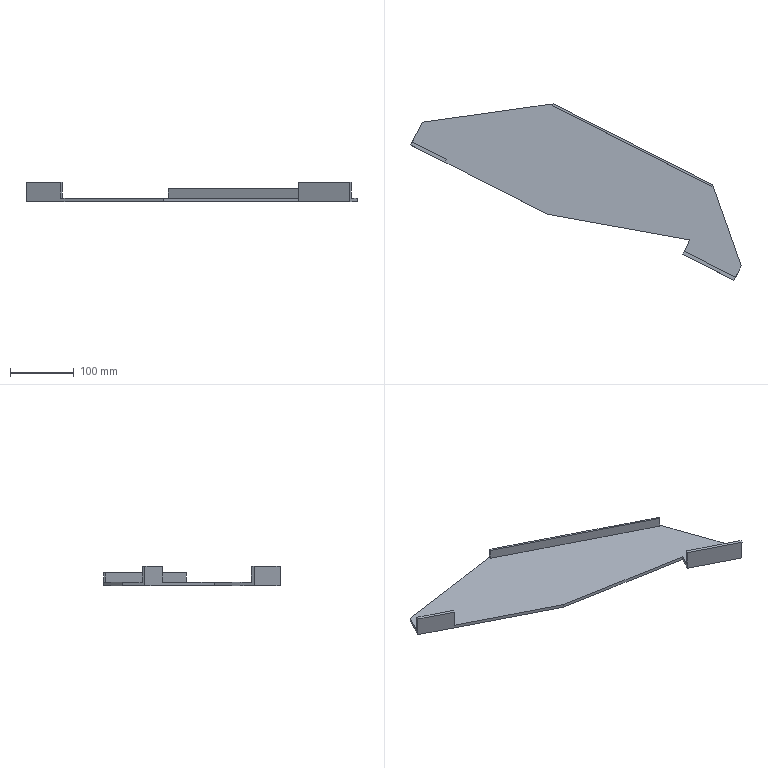Component | SolidWorks | Part18-1 | 2 solids | 22 faces | box 517.58 x 276.19 x 30 mm | volume 338137 mm3 | plane 22
build123d program:
from build123d import *

# Parameters (mm, degrees)
BOSS_EXTRUDE1_DEPTH = 5
SKETCH2_W           = 90
SKETCH2_H           = 30
BOSS_EXTRUDE2_DEPTH = 5
SKETCH3_W           = 280
SKETCH3_H           = 15
BOSS_EXTRUDE3_DEPTH = 3
SKETCH4_W           = 60
SKETCH4_H           = 25
BOSS_EXTRUDE4_DEPTH = 5


with BuildPart() as part:
    # Sketch1 → Boss-Extrude1 (new body)
    with BuildSketch(Plane.XY):
        Polygon((-37.937, 0), (-37.937, 20), (59.702, 113.229), (339.702, 113.229), (509.386, -5), (509.386, -45), (269.386, -45), (52.063, 20), (52.063, 0), align=None)
    extrude(amount=BOSS_EXTRUDE1_DEPTH)

    # Sketch2 → Boss-Extrude2 (add)
    with BuildSketch(Plane(origin=(0, 0, 0), x_dir=(-1, 0, 0), z_dir=(0, -1, 0))):
        with Locations((-7.063, 10)):
            Rectangle(SKETCH2_W, SKETCH2_H)
    extrude(amount=BOSS_EXTRUDE2_DEPTH)

    # Sketch4 → Boss-Extrude4 (add)
    with BuildSketch(Plane(origin=(0, -45, 0), x_dir=(-1, 0, 0), z_dir=(0, -1, 0))):
        with Locations((-479.386, 12.5)):
            Rectangle(SKETCH4_W, SKETCH4_H)
    extrude(amount=-BOSS_EXTRUDE4_DEPTH)


with BuildPart() as body_2:
    # Sketch3 → Boss-Extrude3 (new body)
    with BuildSketch(Plane(origin=(0, 113.229, 0), x_dir=(1, 0, 0), z_dir=(0, 1, 0))):
        with Locations((199.702, 7.5)):
            Rectangle(SKETCH3_W, SKETCH3_H)
    extrude(amount=-BOSS_EXTRUDE3_DEPTH)


solid = Compound([part.part, body_2.part])

# Placed as in the assembly
solid = solid.moved(Location((298.812, -1061.476, 1167.971), (-180, 0, -153.121)))
STEP:
#1=CARTESIAN_POINT('',(11.683,-36.751,45.983));
#2=VERTEX_POINT('',#1);
#3=CARTESIAN_POINT('',(1.85,-31.768,45.983));
#4=VERTEX_POINT('',#3);
#5=CARTESIAN_POINT('',(1.85,-31.768,45.983));
#6=DIRECTION('',(-0.892,0.4521,0.));
#7=VECTOR('',#6,39.37);
#8=LINE('',#5,#7);
#9=EDGE_CURVE('',#2,#4,#8,.T.);
#10=ORIENTED_EDGE('',*,*,#9,.F.);
#11=CARTESIAN_POINT('',(11.63,-36.857,45.983));
#12=VERTEX_POINT('',#11);
#13=CARTESIAN_POINT('',(11.63,-36.857,45.983));
#14=DIRECTION('',(0.4521,0.892,0.));
#15=VECTOR('',#14,39.37);
#16=LINE('',#13,#15);
#17=EDGE_CURVE('',#12,#2,#16,.T.);
#18=ORIENTED_EDGE('',*,*,#17,.F.);
#19=CARTESIAN_POINT('',(1.797,-31.873,45.983));
#20=VERTEX_POINT('',#19);
#21=CARTESIAN_POINT('',(1.797,-31.873,45.983));
#22=DIRECTION('',(-0.892,0.4521,0.));
#23=VECTOR('',#22,39.37);
#24=LINE('',#21,#23);
#25=EDGE_CURVE('',#12,#20,#24,.T.);
#26=ORIENTED_EDGE('',*,*,#25,.T.);
#27=CARTESIAN_POINT('',(1.797,-31.873,45.983));
#28=DIRECTION('',(0.4521,0.892,0.));
#29=VECTOR('',#28,39.37);
#30=LINE('',#27,#29);
#31=EDGE_CURVE('',#20,#4,#30,.T.);
#32=ORIENTED_EDGE('',*,*,#31,.T.);
#33=EDGE_LOOP('',(#10,#18,#26,#32));
#34=FACE_OUTER_BOUND('',#33,.T.);
#35=CARTESIAN_POINT('',(1.797,-31.873,45.983));
#36=DIRECTION('',(0.,0.,-1.));
#37=DIRECTION('',(-0.892,0.4521,0.));
#38=AXIS2_PLACEMENT_3D('',#35,#36,#37);
#39=PLANE('',#38);
#40=ADVANCED_FACE('',(#34),#39,.T.);
#41=CARTESIAN_POINT('',(11.683,-36.751,46.574));
#42=VERTEX_POINT('',#41);
#43=CARTESIAN_POINT('',(11.683,-36.751,45.983));
#44=DIRECTION('',(0.,0.,-1.));
#45=VECTOR('',#44,39.37);
#46=LINE('',#43,#45);
#47=EDGE_CURVE('',#42,#2,#46,.T.);
#48=ORIENTED_EDGE('',*,*,#47,.F.);
#49=CARTESIAN_POINT('',(11.63,-36.857,46.574));
#50=VERTEX_POINT('',#49);
#51=CARTESIAN_POINT('',(11.63,-36.857,46.574));
#52=DIRECTION('',(0.4521,0.892,0.));
#53=VECTOR('',#52,39.37);
#54=LINE('',#51,#53);
#55=EDGE_CURVE('',#50,#42,#54,.T.);
#56=ORIENTED_EDGE('',*,*,#55,.F.);
#57=CARTESIAN_POINT('',(11.63,-36.857,45.983));
#58=DIRECTION('',(0.,0.,-1.));
#59=VECTOR('',#58,39.37);
#60=LINE('',#57,#59);
#61=EDGE_CURVE('',#50,#12,#60,.T.);
#62=ORIENTED_EDGE('',*,*,#61,.T.);
#63=ORIENTED_EDGE('',*,*,#17,.T.);
#64=EDGE_LOOP('',(#48,#56,#62,#63));
#65=FACE_OUTER_BOUND('',#64,.T.);
#66=CARTESIAN_POINT('',(11.63,-36.857,45.983));
#67=DIRECTION('',(0.892,-0.4521,-0.));
#68=DIRECTION('',(0.,0.,-1.));
#69=AXIS2_PLACEMENT_3D('',#66,#67,#68);
#70=PLANE('',#69);
#71=ADVANCED_FACE('',(#65),#70,.T.);
#72=CARTESIAN_POINT('',(1.85,-31.768,46.574));
#73=VERTEX_POINT('',#72);
#74=CARTESIAN_POINT('',(11.683,-36.751,46.574));
#75=DIRECTION('',(0.892,-0.4521,-0.));
#76=VECTOR('',#75,39.37);
#77=LINE('',#74,#76);
#78=EDGE_CURVE('',#73,#42,#77,.T.);
#79=ORIENTED_EDGE('',*,*,#78,.F.);
#80=CARTESIAN_POINT('',(1.797,-31.873,46.574));
#81=VERTEX_POINT('',#80);
#82=CARTESIAN_POINT('',(1.797,-31.873,46.574));
#83=DIRECTION('',(0.4521,0.892,0.));
#84=VECTOR('',#83,39.37);
#85=LINE('',#82,#84);
#86=EDGE_CURVE('',#81,#73,#85,.T.);
#87=ORIENTED_EDGE('',*,*,#86,.F.);
#88=CARTESIAN_POINT('',(11.63,-36.857,46.574));
#89=DIRECTION('',(0.892,-0.4521,-0.));
#90=VECTOR('',#89,39.37);
#91=LINE('',#88,#90);
#92=EDGE_CURVE('',#81,#50,#91,.T.);
#93=ORIENTED_EDGE('',*,*,#92,.T.);
#94=ORIENTED_EDGE('',*,*,#55,.T.);
#95=EDGE_LOOP('',(#79,#87,#93,#94));
#96=FACE_OUTER_BOUND('',#95,.T.);
#97=CARTESIAN_POINT('',(11.63,-36.857,46.574));
#98=DIRECTION('',(-0.,-0.,1.));
#99=DIRECTION('',(0.892,-0.4521,-0.));
#100=AXIS2_PLACEMENT_3D('',#97,#98,#99);
#101=PLANE('',#100);
#102=ADVANCED_FACE('',(#96),#101,.T.);
#103=CARTESIAN_POINT('',(1.85,-31.768,46.574));
#104=DIRECTION('',(-0.,-0.,1.));
#105=VECTOR('',#104,39.37);
#106=LINE('',#103,#105);
#107=EDGE_CURVE('',#4,#73,#106,.T.);
#108=ORIENTED_EDGE('',*,*,#107,.F.);
#109=ORIENTED_EDGE('',*,*,#31,.F.);
#110=CARTESIAN_POINT('',(1.797,-31.873,46.574));
#111=DIRECTION('',(-0.,-0.,1.));
#112=VECTOR('',#111,39.37);
#113=LINE('',#110,#112);
#114=EDGE_CURVE('',#20,#81,#113,.T.);
#115=ORIENTED_EDGE('',*,*,#114,.T.);
#116=ORIENTED_EDGE('',*,*,#86,.T.);
#117=EDGE_LOOP('',(#108,#109,#115,#116));
#118=FACE_OUTER_BOUND('',#117,.T.);
#119=CARTESIAN_POINT('',(1.797,-31.873,46.574));
#120=DIRECTION('',(-0.892,0.4521,0.));
#121=DIRECTION('',(-0.,-0.,1.));
#122=AXIS2_PLACEMENT_3D('',#119,#120,#121);
#123=PLANE('',#122);
#124=ADVANCED_FACE('',(#118),#123,.T.);
#125=ORIENTED_EDGE('',*,*,#25,.F.);
#126=ORIENTED_EDGE('',*,*,#61,.F.);
#127=ORIENTED_EDGE('',*,*,#92,.F.);
#128=ORIENTED_EDGE('',*,*,#114,.F.);
#129=EDGE_LOOP('',(#125,#126,#127,#128));
#130=FACE_OUTER_BOUND('',#129,.T.);
#131=CARTESIAN_POINT('',(13.726,-37.919,45.983));
#132=DIRECTION('',(-0.4521,-0.892,-0.));
#133=DIRECTION('',(-0.,-0.,1.));
#134=AXIS2_PLACEMENT_3D('',#131,#132,#133);
#135=PLANE('',#134);
#136=ADVANCED_FACE('',(#130),#135,.T.);
#137=ORIENTED_EDGE('',*,*,#9,.T.);
#138=ORIENTED_EDGE('',*,*,#107,.T.);
#139=ORIENTED_EDGE('',*,*,#78,.T.);
#140=ORIENTED_EDGE('',*,*,#47,.T.);
#141=EDGE_LOOP('',(#137,#138,#139,#140));
#142=FACE_OUTER_BOUND('',#141,.T.);
#143=CARTESIAN_POINT('',(13.78,-37.814,45.983));
#144=DIRECTION('',(-0.4521,-0.892,-0.));
#145=DIRECTION('',(-0.,-0.,1.));
#146=AXIS2_PLACEMENT_3D('',#143,#144,#145);
#147=PLANE('',#146);
#148=ADVANCED_FACE('',(#142),#147,.F.);
#149=CLOSED_SHELL('',(#40,#71,#102,#124,#136,#148));
#150=MANIFOLD_SOLID_BREP('',#149);
#151=CARTESIAN_POINT('',(9.936,-40.864,45.983));
#152=VERTEX_POINT('',#151);
#153=CARTESIAN_POINT('',(10.292,-40.161,45.983));
#154=VERTEX_POINT('',#153);
#155=CARTESIAN_POINT('',(9.936,-40.864,45.983));
#156=DIRECTION('',(0.4521,0.892,0.));
#157=VECTOR('',#156,39.37);
#158=LINE('',#155,#157);
#159=EDGE_CURVE('',#152,#154,#158,.T.);
#160=ORIENTED_EDGE('',*,*,#159,.T.);
#161=CARTESIAN_POINT('',(10.292,-40.161,45.786));
#162=VERTEX_POINT('',#161);
#163=CARTESIAN_POINT('',(10.292,-40.161,45.786));
#164=DIRECTION('',(-0.,-0.,1.));
#165=VECTOR('',#164,39.37);
#166=LINE('',#163,#165);
#167=EDGE_CURVE('',#162,#154,#166,.T.);
#168=ORIENTED_EDGE('',*,*,#167,.F.);
#169=CARTESIAN_POINT('',(9.847,-41.039,45.786));
#170=VERTEX_POINT('',#169);
#171=CARTESIAN_POINT('',(9.936,-40.864,45.786));
#172=DIRECTION('',(0.4521,0.892,0.));
#173=VECTOR('',#172,39.37);
#174=LINE('',#171,#173);
#175=EDGE_CURVE('',#170,#162,#174,.T.);
#176=ORIENTED_EDGE('',*,*,#175,.F.);
#177=CARTESIAN_POINT('',(9.847,-41.039,46.967));
#178=VERTEX_POINT('',#177);
#179=CARTESIAN_POINT('',(9.847,-41.039,45.786));
#180=DIRECTION('',(0.,0.,-1.));
#181=VECTOR('',#180,39.37);
#182=LINE('',#179,#181);
#183=EDGE_CURVE('',#178,#170,#182,.T.);
#184=ORIENTED_EDGE('',*,*,#183,.F.);
#185=CARTESIAN_POINT('',(9.936,-40.864,46.967));
#186=VERTEX_POINT('',#185);
#187=CARTESIAN_POINT('',(9.847,-41.039,46.967));
#188=DIRECTION('',(0.4521,0.892,0.));
#189=VECTOR('',#188,39.37);
#190=LINE('',#187,#189);
#191=EDGE_CURVE('',#178,#186,#190,.T.);
#192=ORIENTED_EDGE('',*,*,#191,.T.);
#193=CARTESIAN_POINT('',(9.936,-40.864,45.786));
#194=DIRECTION('',(0.,0.,-1.));
#195=VECTOR('',#194,39.37);
#196=LINE('',#193,#195);
#197=EDGE_CURVE('',#186,#152,#196,.T.);
#198=ORIENTED_EDGE('',*,*,#197,.T.);
#199=EDGE_LOOP('',(#160,#168,#176,#184,#192,#198));
#200=FACE_OUTER_BOUND('',#199,.T.);
#201=CARTESIAN_POINT('',(9.936,-40.864,45.786));
#202=DIRECTION('',(0.892,-0.4521,-0.));
#203=DIRECTION('',(0.,0.,-1.));
#204=AXIS2_PLACEMENT_3D('',#201,#202,#203);
#205=PLANE('',#204);
#206=ADVANCED_FACE('',(#200),#205,.F.);
#207=CARTESIAN_POINT('',(1.503,-38.576,45.983));
#208=VERTEX_POINT('',#207);
#209=CARTESIAN_POINT('',(10.292,-40.161,45.983));
#210=DIRECTION('',(-0.9841,0.1775,0.));
#211=VECTOR('',#210,39.37);
#212=LINE('',#209,#211);
#213=EDGE_CURVE('',#154,#208,#212,.T.);
#214=ORIENTED_EDGE('',*,*,#213,.T.);
#215=CARTESIAN_POINT('',(1.503,-38.576,45.786));
#216=VERTEX_POINT('',#215);
#217=CARTESIAN_POINT('',(1.503,-38.576,45.786));
#218=DIRECTION('',(-0.,-0.,1.));
#219=VECTOR('',#218,39.37);
#220=LINE('',#217,#219);
#221=EDGE_CURVE('',#216,#208,#220,.T.);
#222=ORIENTED_EDGE('',*,*,#221,.F.);
#223=CARTESIAN_POINT('',(10.292,-40.161,45.786));
#224=DIRECTION('',(-0.9841,0.1775,0.));
#225=VECTOR('',#224,39.37);
#226=LINE('',#223,#225);
#227=EDGE_CURVE('',#162,#216,#226,.T.);
#228=ORIENTED_EDGE('',*,*,#227,.F.);
#229=ORIENTED_EDGE('',*,*,#167,.T.);
#230=EDGE_LOOP('',(#214,#222,#228,#229));
#231=FACE_OUTER_BOUND('',#230,.T.);
#232=CARTESIAN_POINT('',(10.292,-40.161,45.786));
#233=DIRECTION('',(0.1775,0.9841,0.));
#234=DIRECTION('',(0.9841,-0.1775,-0.));
#235=AXIS2_PLACEMENT_3D('',#232,#233,#234);
#236=PLANE('',#235);
#237=ADVANCED_FACE('',(#231),#236,.F.);
#238=CARTESIAN_POINT('',(-4.818,-35.372,45.983));
#239=VERTEX_POINT('',#238);
#240=CARTESIAN_POINT('',(1.503,-38.576,45.983));
#241=DIRECTION('',(-0.892,0.4521,0.));
#242=VECTOR('',#241,39.37);
#243=LINE('',#240,#242);
#244=EDGE_CURVE('',#208,#239,#243,.T.);
#245=ORIENTED_EDGE('',*,*,#244,.T.);
#246=CARTESIAN_POINT('',(-4.818,-35.372,46.967));
#247=VERTEX_POINT('',#246);
#248=CARTESIAN_POINT('',(-4.818,-35.372,46.967));
#249=DIRECTION('',(-0.,-0.,1.));
#250=VECTOR('',#249,39.37);
#251=LINE('',#248,#250);
#252=EDGE_CURVE('',#239,#247,#251,.T.);
#253=ORIENTED_EDGE('',*,*,#252,.T.);
#254=CARTESIAN_POINT('',(-6.925,-34.304,46.967));
#255=VERTEX_POINT('',#254);
#256=CARTESIAN_POINT('',(-6.925,-34.304,46.967));
#257=DIRECTION('',(-0.892,0.4521,0.));
#258=VECTOR('',#257,39.37);
#259=LINE('',#256,#258);
#260=EDGE_CURVE('',#247,#255,#259,.T.);
#261=ORIENTED_EDGE('',*,*,#260,.T.);
#262=CARTESIAN_POINT('',(-6.925,-34.304,45.786));
#263=VERTEX_POINT('',#262);
#264=CARTESIAN_POINT('',(-6.925,-34.304,45.786));
#265=DIRECTION('',(-0.,-0.,1.));
#266=VECTOR('',#265,39.37);
#267=LINE('',#264,#266);
#268=EDGE_CURVE('',#263,#255,#267,.T.);
#269=ORIENTED_EDGE('',*,*,#268,.F.);
#270=CARTESIAN_POINT('',(1.503,-38.576,45.786));
#271=DIRECTION('',(-0.892,0.4521,0.));
#272=VECTOR('',#271,39.37);
#273=LINE('',#270,#272);
#274=EDGE_CURVE('',#216,#263,#273,.T.);
#275=ORIENTED_EDGE('',*,*,#274,.F.);
#276=ORIENTED_EDGE('',*,*,#221,.T.);
#277=EDGE_LOOP('',(#245,#253,#261,#269,#275,#276));
#278=FACE_OUTER_BOUND('',#277,.T.);
#279=CARTESIAN_POINT('',(1.503,-38.576,45.786));
#280=DIRECTION('',(0.4521,0.892,0.));
#281=DIRECTION('',(0.,0.,-1.));
#282=AXIS2_PLACEMENT_3D('',#279,#280,#281);
#283=PLANE('',#282);
#284=ADVANCED_FACE('',(#278),#283,.F.);
#285=ORIENTED_EDGE('',*,*,#268,.T.);
#286=CARTESIAN_POINT('',(-6.836,-34.128,46.967));
#287=VERTEX_POINT('',#286);
#288=CARTESIAN_POINT('',(-6.836,-34.128,46.967));
#289=DIRECTION('',(-0.4521,-0.892,-0.));
#290=VECTOR('',#289,39.37);
#291=LINE('',#288,#290);
#292=EDGE_CURVE('',#287,#255,#291,.T.);
#293=ORIENTED_EDGE('',*,*,#292,.F.);
#294=CARTESIAN_POINT('',(-6.836,-34.128,45.983));
#295=VERTEX_POINT('',#294);
#296=CARTESIAN_POINT('',(-6.836,-34.128,45.983));
#297=DIRECTION('',(0.,0.,-1.));
#298=VECTOR('',#297,39.37);
#299=LINE('',#296,#298);
#300=EDGE_CURVE('',#287,#295,#299,.T.);
#301=ORIENTED_EDGE('',*,*,#300,.T.);
#302=CARTESIAN_POINT('',(-6.213,-32.899,45.983));
#303=VERTEX_POINT('',#302);
#304=CARTESIAN_POINT('',(-6.925,-34.304,45.983));
#305=DIRECTION('',(0.4521,0.892,0.));
#306=VECTOR('',#305,39.37);
#307=LINE('',#304,#306);
#308=EDGE_CURVE('',#295,#303,#307,.T.);
#309=ORIENTED_EDGE('',*,*,#308,.T.);
#310=CARTESIAN_POINT('',(-6.213,-32.899,45.786));
#311=VERTEX_POINT('',#310);
#312=CARTESIAN_POINT('',(-6.213,-32.899,45.786));
#313=DIRECTION('',(-0.,-0.,1.));
#314=VECTOR('',#313,39.37);
#315=LINE('',#312,#314);
#316=EDGE_CURVE('',#311,#303,#315,.T.);
#317=ORIENTED_EDGE('',*,*,#316,.F.);
#318=CARTESIAN_POINT('',(-6.925,-34.304,45.786));
#319=DIRECTION('',(0.4521,0.892,0.));
#320=VECTOR('',#319,39.37);
#321=LINE('',#318,#320);
#322=EDGE_CURVE('',#263,#311,#321,.T.);
#323=ORIENTED_EDGE('',*,*,#322,.F.);
#324=EDGE_LOOP('',(#285,#293,#301,#309,#317,#323));
#325=FACE_OUTER_BOUND('',#324,.T.);
#326=CARTESIAN_POINT('',(-6.925,-34.304,45.786));
#327=DIRECTION('',(0.892,-0.4521,-0.));
#328=DIRECTION('',(0.,0.,-1.));
#329=AXIS2_PLACEMENT_3D('',#326,#327,#328);
#330=PLANE('',#329);
#331=ADVANCED_FACE('',(#325),#330,.F.);
#332=CARTESIAN_POINT('',(1.85,-31.768,45.983));
#333=VERTEX_POINT('',#332);
#334=CARTESIAN_POINT('',(-6.213,-32.899,45.983));
#335=DIRECTION('',(0.9903,0.139,0.));
#336=VECTOR('',#335,39.37);
#337=LINE('',#334,#336);
#338=EDGE_CURVE('',#303,#333,#337,.T.);
#339=ORIENTED_EDGE('',*,*,#338,.T.);
#340=CARTESIAN_POINT('',(1.85,-31.768,45.786));
#341=VERTEX_POINT('',#340);
#342=CARTESIAN_POINT('',(1.85,-31.768,45.786));
#343=DIRECTION('',(-0.,-0.,1.));
#344=VECTOR('',#343,39.37);
#345=LINE('',#342,#344);
#346=EDGE_CURVE('',#341,#333,#345,.T.);
#347=ORIENTED_EDGE('',*,*,#346,.F.);
#348=CARTESIAN_POINT('',(-6.213,-32.899,45.786));
#349=DIRECTION('',(0.9903,0.139,0.));
#350=VECTOR('',#349,39.37);
#351=LINE('',#348,#350);
#352=EDGE_CURVE('',#311,#341,#351,.T.);
#353=ORIENTED_EDGE('',*,*,#352,.F.);
#354=ORIENTED_EDGE('',*,*,#316,.T.);
#355=EDGE_LOOP('',(#339,#347,#353,#354));
#356=FACE_OUTER_BOUND('',#355,.T.);
#357=CARTESIAN_POINT('',(-6.213,-32.899,45.786));
#358=DIRECTION('',(0.139,-0.9903,-0.));
#359=DIRECTION('',(-0.9903,-0.139,-0.));
#360=AXIS2_PLACEMENT_3D('',#357,#358,#359);
#361=PLANE('',#360);
#362=ADVANCED_FACE('',(#356),#361,.F.);
#363=CARTESIAN_POINT('',(11.683,-36.751,45.983));
#364=VERTEX_POINT('',#363);
#365=CARTESIAN_POINT('',(11.683,-36.751,45.983));
#366=DIRECTION('',(0.892,-0.4521,-0.));
#367=VECTOR('',#366,39.37);
#368=LINE('',#365,#367);
#369=EDGE_CURVE('',#333,#364,#368,.T.);
#370=ORIENTED_EDGE('',*,*,#369,.T.);
#371=CARTESIAN_POINT('',(11.683,-36.751,45.786));
#372=VERTEX_POINT('',#371);
#373=CARTESIAN_POINT('',(11.683,-36.751,45.786));
#374=DIRECTION('',(-0.,-0.,1.));
#375=VECTOR('',#374,39.37);
#376=LINE('',#373,#375);
#377=EDGE_CURVE('',#372,#364,#376,.T.);
#378=ORIENTED_EDGE('',*,*,#377,.F.);
#379=CARTESIAN_POINT('',(11.683,-36.751,45.786));
#380=DIRECTION('',(0.892,-0.4521,-0.));
#381=VECTOR('',#380,39.37);
#382=LINE('',#379,#381);
#383=EDGE_CURVE('',#341,#372,#382,.T.);
#384=ORIENTED_EDGE('',*,*,#383,.F.);
#385=ORIENTED_EDGE('',*,*,#346,.T.);
#386=EDGE_LOOP('',(#370,#378,#384,#385));
#387=FACE_OUTER_BOUND('',#386,.T.);
#388=CARTESIAN_POINT('',(11.683,-36.751,45.786));
#389=DIRECTION('',(-0.4521,-0.892,-0.));
#390=DIRECTION('',(-0.,-0.,1.));
#391=AXIS2_PLACEMENT_3D('',#388,#389,#390);
#392=PLANE('',#391);
#393=ADVANCED_FACE('',(#387),#392,.F.);
#394=CARTESIAN_POINT('',(13.452,-41.763,45.983));
#395=VERTEX_POINT('',#394);
#396=CARTESIAN_POINT('',(13.452,-41.763,45.983));
#397=DIRECTION('',(0.3329,-0.943,-0.));
#398=VECTOR('',#397,39.37);
#399=LINE('',#396,#398);
#400=EDGE_CURVE('',#364,#395,#399,.T.);
#401=ORIENTED_EDGE('',*,*,#400,.T.);
#402=CARTESIAN_POINT('',(13.452,-41.763,45.786));
#403=VERTEX_POINT('',#402);
#404=CARTESIAN_POINT('',(13.452,-41.763,45.786));
#405=DIRECTION('',(-0.,-0.,1.));
#406=VECTOR('',#405,39.37);
#407=LINE('',#404,#406);
#408=EDGE_CURVE('',#403,#395,#407,.T.);
#409=ORIENTED_EDGE('',*,*,#408,.F.);
#410=CARTESIAN_POINT('',(13.452,-41.763,45.786));
#411=DIRECTION('',(0.3329,-0.943,-0.));
#412=VECTOR('',#411,39.37);
#413=LINE('',#410,#412);
#414=EDGE_CURVE('',#372,#403,#413,.T.);
#415=ORIENTED_EDGE('',*,*,#414,.F.);
#416=ORIENTED_EDGE('',*,*,#377,.T.);
#417=EDGE_LOOP('',(#401,#409,#415,#416));
#418=FACE_OUTER_BOUND('',#417,.T.);
#419=CARTESIAN_POINT('',(13.452,-41.763,45.786));
#420=DIRECTION('',(-0.943,-0.3329,-0.));
#421=DIRECTION('',(-0.3329,0.943,0.));
#422=AXIS2_PLACEMENT_3D('',#419,#420,#421);
#423=PLANE('',#422);
#424=ADVANCED_FACE('',(#418),#423,.F.);
#425=CARTESIAN_POINT('',(13.096,-42.466,45.983));
#426=VERTEX_POINT('',#425);
#427=CARTESIAN_POINT('',(13.096,-42.466,45.983));
#428=DIRECTION('',(-0.4521,-0.892,-0.));
#429=VECTOR('',#428,39.37);
#430=LINE('',#427,#429);
#431=EDGE_CURVE('',#395,#426,#430,.T.);
#432=ORIENTED_EDGE('',*,*,#431,.T.);
#433=CARTESIAN_POINT('',(13.096,-42.466,46.967));
#434=VERTEX_POINT('',#433);
#435=CARTESIAN_POINT('',(13.096,-42.466,46.967));
#436=DIRECTION('',(-0.,-0.,1.));
#437=VECTOR('',#436,39.37);
#438=LINE('',#435,#437);
#439=EDGE_CURVE('',#426,#434,#438,.T.);
#440=ORIENTED_EDGE('',*,*,#439,.T.);
#441=CARTESIAN_POINT('',(13.007,-42.641,46.967));
#442=VERTEX_POINT('',#441);
#443=CARTESIAN_POINT('',(13.007,-42.641,46.967));
#444=DIRECTION('',(0.4521,0.892,0.));
#445=VECTOR('',#444,39.37);
#446=LINE('',#443,#445);
#447=EDGE_CURVE('',#442,#434,#446,.T.);
#448=ORIENTED_EDGE('',*,*,#447,.F.);
#449=CARTESIAN_POINT('',(13.007,-42.641,45.786));
#450=VERTEX_POINT('',#449);
#451=CARTESIAN_POINT('',(13.007,-42.641,46.967));
#452=DIRECTION('',(-0.,-0.,1.));
#453=VECTOR('',#452,39.37);
#454=LINE('',#451,#453);
#455=EDGE_CURVE('',#450,#442,#454,.T.);
#456=ORIENTED_EDGE('',*,*,#455,.F.);
#457=CARTESIAN_POINT('',(13.096,-42.466,45.786));
#458=DIRECTION('',(-0.4521,-0.892,-0.));
#459=VECTOR('',#458,39.37);
#460=LINE('',#457,#459);
#461=EDGE_CURVE('',#403,#450,#460,.T.);
#462=ORIENTED_EDGE('',*,*,#461,.F.);
#463=ORIENTED_EDGE('',*,*,#408,.T.);
#464=EDGE_LOOP('',(#432,#440,#448,#456,#462,#463));
#465=FACE_OUTER_BOUND('',#464,.T.);
#466=CARTESIAN_POINT('',(13.096,-42.466,45.786));
#467=DIRECTION('',(-0.892,0.4521,0.));
#468=DIRECTION('',(-0.,-0.,1.));
#469=AXIS2_PLACEMENT_3D('',#466,#467,#468);
#470=PLANE('',#469);
#471=ADVANCED_FACE('',(#465),#470,.F.);
#472=ORIENTED_EDGE('',*,*,#461,.T.);
#473=CARTESIAN_POINT('',(13.007,-42.641,45.786));
#474=DIRECTION('',(0.892,-0.4521,-0.));
#475=VECTOR('',#474,39.37);
#476=LINE('',#473,#475);
#477=EDGE_CURVE('',#170,#450,#476,.T.);
#478=ORIENTED_EDGE('',*,*,#477,.F.);
#479=ORIENTED_EDGE('',*,*,#175,.T.);
#480=ORIENTED_EDGE('',*,*,#227,.T.);
#481=ORIENTED_EDGE('',*,*,#274,.T.);
#482=ORIENTED_EDGE('',*,*,#322,.T.);
#483=ORIENTED_EDGE('',*,*,#352,.T.);
#484=ORIENTED_EDGE('',*,*,#383,.T.);
#485=ORIENTED_EDGE('',*,*,#414,.T.);
#486=EDGE_LOOP('',(#472,#478,#479,#480,#481,#482,#483,#484,#485));
#487=FACE_OUTER_BOUND('',#486,.T.);
#488=CARTESIAN_POINT('',(11.764,-41.79,45.786));
#489=DIRECTION('',(0.,0.,-1.));
#490=DIRECTION('',(-0.892,0.4521,0.));
#491=AXIS2_PLACEMENT_3D('',#488,#489,#490);
#492=PLANE('',#491);
#493=ADVANCED_FACE('',(#487),#492,.T.);
#494=CARTESIAN_POINT('',(-4.729,-35.196,45.983));
#495=VERTEX_POINT('',#494);
#496=CARTESIAN_POINT('',(-4.729,-35.196,45.983));
#497=DIRECTION('',(0.892,-0.4521,-0.));
#498=VECTOR('',#497,39.37);
#499=LINE('',#496,#498);
#500=EDGE_CURVE('',#295,#495,#499,.T.);
#501=ORIENTED_EDGE('',*,*,#500,.T.);
#502=CARTESIAN_POINT('',(-4.729,-35.196,45.983));
#503=DIRECTION('',(-0.4521,-0.892,-0.));
#504=VECTOR('',#503,39.37);
#505=LINE('',#502,#504);
#506=EDGE_CURVE('',#495,#239,#505,.T.);
#507=ORIENTED_EDGE('',*,*,#506,.T.);
#508=ORIENTED_EDGE('',*,*,#244,.F.);
#509=ORIENTED_EDGE('',*,*,#213,.F.);
#510=ORIENTED_EDGE('',*,*,#159,.F.);
#511=CARTESIAN_POINT('',(13.096,-42.466,45.983));
#512=DIRECTION('',(-0.892,0.4521,0.));
#513=VECTOR('',#512,39.37);
#514=LINE('',#511,#513);
#515=EDGE_CURVE('',#426,#152,#514,.T.);
#516=ORIENTED_EDGE('',*,*,#515,.F.);
#517=ORIENTED_EDGE('',*,*,#431,.F.);
#518=ORIENTED_EDGE('',*,*,#400,.F.);
#519=ORIENTED_EDGE('',*,*,#369,.F.);
#520=ORIENTED_EDGE('',*,*,#338,.F.);
#521=ORIENTED_EDGE('',*,*,#308,.F.);
#522=EDGE_LOOP('',(#501,#507,#508,#509,#510,#516,#517,#518,#519,#520,#521));
#523=FACE_OUTER_BOUND('',#522,.T.);
#524=CARTESIAN_POINT('',(11.764,-41.79,45.983));
#525=DIRECTION('',(0.,0.,-1.));
#526=DIRECTION('',(-0.892,0.4521,0.));
#527=AXIS2_PLACEMENT_3D('',#524,#525,#526);
#528=PLANE('',#527);
#529=ADVANCED_FACE('',(#523),#528,.F.);
#530=ORIENTED_EDGE('',*,*,#515,.T.);
#531=ORIENTED_EDGE('',*,*,#197,.F.);
#532=CARTESIAN_POINT('',(9.936,-40.864,46.967));
#533=DIRECTION('',(-0.892,0.4521,0.));
#534=VECTOR('',#533,39.37);
#535=LINE('',#532,#534);
#536=EDGE_CURVE('',#434,#186,#535,.T.);
#537=ORIENTED_EDGE('',*,*,#536,.F.);
#538=ORIENTED_EDGE('',*,*,#439,.F.);
#539=EDGE_LOOP('',(#530,#531,#537,#538));
#540=FACE_OUTER_BOUND('',#539,.T.);
#541=CARTESIAN_POINT('',(11.764,-41.79,45.983));
#542=DIRECTION('',(0.4521,0.892,0.));
#543=DIRECTION('',(0.,0.,-1.));
#544=AXIS2_PLACEMENT_3D('',#541,#542,#543);
#545=PLANE('',#544);
#546=ADVANCED_FACE('',(#540),#545,.T.);
#547=ORIENTED_EDGE('',*,*,#536,.T.);
#548=ORIENTED_EDGE('',*,*,#191,.F.);
#549=CARTESIAN_POINT('',(9.847,-41.039,46.967));
#550=DIRECTION('',(-0.892,0.4521,0.));
#551=VECTOR('',#550,39.37);
#552=LINE('',#549,#551);
#553=EDGE_CURVE('',#442,#178,#552,.T.);
#554=ORIENTED_EDGE('',*,*,#553,.F.);
#555=ORIENTED_EDGE('',*,*,#447,.T.);
#556=EDGE_LOOP('',(#547,#548,#554,#555));
#557=FACE_OUTER_BOUND('',#556,.T.);
#558=CARTESIAN_POINT('',(9.847,-41.039,46.967));
#559=DIRECTION('',(0.,0.,-1.));
#560=DIRECTION('',(-0.892,0.4521,0.));
#561=AXIS2_PLACEMENT_3D('',#558,#559,#560);
#562=PLANE('',#561);
#563=ADVANCED_FACE('',(#557),#562,.F.);
#564=ORIENTED_EDGE('',*,*,#455,.T.);
#565=ORIENTED_EDGE('',*,*,#553,.T.);
#566=ORIENTED_EDGE('',*,*,#183,.T.);
#567=ORIENTED_EDGE('',*,*,#477,.T.);
#568=EDGE_LOOP('',(#564,#565,#566,#567));
#569=FACE_OUTER_BOUND('',#568,.T.);
#570=CARTESIAN_POINT('',(11.675,-41.966,45.983));
#571=DIRECTION('',(0.4521,0.892,0.));
#572=DIRECTION('',(0.,0.,-1.));
#573=AXIS2_PLACEMENT_3D('',#570,#571,#572);
#574=PLANE('',#573);
#575=ADVANCED_FACE('',(#569),#574,.F.);
#576=ORIENTED_EDGE('',*,*,#260,.F.);
#577=CARTESIAN_POINT('',(-4.729,-35.196,46.967));
#578=VERTEX_POINT('',#577);
#579=CARTESIAN_POINT('',(-4.729,-35.196,46.967));
#580=DIRECTION('',(-0.4521,-0.892,-0.));
#581=VECTOR('',#580,39.37);
#582=LINE('',#579,#581);
#583=EDGE_CURVE('',#578,#247,#582,.T.);
#584=ORIENTED_EDGE('',*,*,#583,.F.);
#585=CARTESIAN_POINT('',(-6.836,-34.128,46.967));
#586=DIRECTION('',(-0.892,0.4521,0.));
#587=VECTOR('',#586,39.37);
#588=LINE('',#585,#587);
#589=EDGE_CURVE('',#578,#287,#588,.T.);
#590=ORIENTED_EDGE('',*,*,#589,.T.);
#591=ORIENTED_EDGE('',*,*,#292,.T.);
#592=EDGE_LOOP('',(#576,#584,#590,#591));
#593=FACE_OUTER_BOUND('',#592,.T.);
#594=CARTESIAN_POINT('',(-6.836,-34.128,46.967));
#595=DIRECTION('',(-0.,-0.,1.));
#596=DIRECTION('',(0.892,-0.4521,-0.));
#597=AXIS2_PLACEMENT_3D('',#594,#595,#596);
#598=PLANE('',#597);
#599=ADVANCED_FACE('',(#593),#598,.T.);
#600=ORIENTED_EDGE('',*,*,#252,.F.);
#601=ORIENTED_EDGE('',*,*,#506,.F.);
#602=CARTESIAN_POINT('',(-4.729,-35.196,46.967));
#603=DIRECTION('',(-0.,-0.,1.));
#604=VECTOR('',#603,39.37);
#605=LINE('',#602,#604);
#606=EDGE_CURVE('',#495,#578,#605,.T.);
#607=ORIENTED_EDGE('',*,*,#606,.T.);
#608=ORIENTED_EDGE('',*,*,#583,.T.);
#609=EDGE_LOOP('',(#600,#601,#607,#608));
#610=FACE_OUTER_BOUND('',#609,.T.);
#611=CARTESIAN_POINT('',(-4.729,-35.196,46.967));
#612=DIRECTION('',(0.892,-0.4521,-0.));
#613=DIRECTION('',(0.,0.,-1.));
#614=AXIS2_PLACEMENT_3D('',#611,#612,#613);
#615=PLANE('',#614);
#616=ADVANCED_FACE('',(#610),#615,.T.);
#617=ORIENTED_EDGE('',*,*,#500,.F.);
#618=ORIENTED_EDGE('',*,*,#300,.F.);
#619=ORIENTED_EDGE('',*,*,#589,.F.);
#620=ORIENTED_EDGE('',*,*,#606,.F.);
#621=EDGE_LOOP('',(#617,#618,#619,#620));
#622=FACE_OUTER_BOUND('',#621,.T.);
#623=CARTESIAN_POINT('',(11.052,-43.195,45.983));
#624=DIRECTION('',(0.4521,0.892,0.));
#625=DIRECTION('',(0.,0.,-1.));
#626=AXIS2_PLACEMENT_3D('',#623,#624,#625);
#627=PLANE('',#626);
#628=ADVANCED_FACE('',(#622),#627,.T.);
#629=CLOSED_SHELL('',(#206,#237,#284,#331,#362,#393,#424,#471,#493,#529,#546,#563,#575,#599,#616,#628));
#630=MANIFOLD_SOLID_BREP('',#629);
#631=CARTESIAN_POINT('',(0.,0.,0.));
#632=DIRECTION('',(0.,0.,1.));
#633=DIRECTION('',(1.,0.,0.));
#634=AXIS2_PLACEMENT_3D('',#631,#632,#633);
#635=(LENGTH_UNIT()NAMED_UNIT(*)SI_UNIT($,.METRE.));
#636=LENGTH_MEASURE_WITH_UNIT(LENGTH_MEASURE(0.0254),#635);
#637=DIMENSIONAL_EXPONENTS(1.,0.,0.,0.,0.,0.,0.);
#638=(CONVERSION_BASED_UNIT('',#636)LENGTH_UNIT()NAMED_UNIT(#637));
#639=UNCERTAINTY_MEASURE_WITH_UNIT(LENGTH_MEASURE(0.00001),#638,'','');
#640=(NAMED_UNIT(*)PLANE_ANGLE_UNIT()SI_UNIT($,.RADIAN.));
#641=(NAMED_UNIT(*)SI_UNIT($,.STERADIAN.)SOLID_ANGLE_UNIT());
#642=(GEOMETRIC_REPRESENTATION_CONTEXT(3)GLOBAL_UNCERTAINTY_ASSIGNED_CONTEXT((#639))GLOBAL_UNIT_ASSIGNED_CONTEXT((#638,#640,#641))REPRESENTATION_CONTEXT('',''));
#643=ADVANCED_BREP_SHAPE_REPRESENTATION('',(#150,#630,#634),#642);
#644=COLOUR_RGB('',0.7922,0.8196,0.9333);
#645=FILL_AREA_STYLE_COLOUR('',#644);
#646=FILL_AREA_STYLE('',(#645));
#647=SURFACE_STYLE_FILL_AREA(#646);
#648=SURFACE_SIDE_STYLE('',(#647));
#649=SURFACE_STYLE_USAGE(.BOTH.,#648);
#650=PRESENTATION_STYLE_ASSIGNMENT((#649));
#651=STYLED_ITEM('',(#650),#630);
#652=PRESENTATION_LAYER_ASSIGNMENT('','',(#651));
#653=(LENGTH_UNIT()NAMED_UNIT(*)SI_UNIT($,.METRE.));
#654=LENGTH_MEASURE_WITH_UNIT(LENGTH_MEASURE(0.0254),#653);
#655=DIMENSIONAL_EXPONENTS(1.,0.,0.,0.,0.,0.,0.);
#656=(CONVERSION_BASED_UNIT('',#654)LENGTH_UNIT()NAMED_UNIT(#655));
#657=UNCERTAINTY_MEASURE_WITH_UNIT(LENGTH_MEASURE(0.00001),#656,'','');
#658=(NAMED_UNIT(*)PLANE_ANGLE_UNIT()SI_UNIT($,.RADIAN.));
#659=(NAMED_UNIT(*)SI_UNIT($,.STERADIAN.)SOLID_ANGLE_UNIT());
#660=(GEOMETRIC_REPRESENTATION_CONTEXT(3)GLOBAL_UNCERTAINTY_ASSIGNED_CONTEXT((#657))GLOBAL_UNIT_ASSIGNED_CONTEXT((#656,#658,#659))REPRESENTATION_CONTEXT('',''));
#661=MECHANICAL_DESIGN_GEOMETRIC_PRESENTATION_REPRESENTATION('',(#651),#660);
#662=COLOUR_RGB('',0.7922,0.8196,0.9333);
#663=FILL_AREA_STYLE_COLOUR('',#662);
#664=FILL_AREA_STYLE('',(#663));
#665=SURFACE_STYLE_FILL_AREA(#664);
#666=SURFACE_SIDE_STYLE('',(#665));
#667=SURFACE_STYLE_USAGE(.BOTH.,#666);
#668=PRESENTATION_STYLE_ASSIGNMENT((#667));
#669=STYLED_ITEM('',(#668),#150);
#670=PRESENTATION_LAYER_ASSIGNMENT('','',(#669));
#671=(LENGTH_UNIT()NAMED_UNIT(*)SI_UNIT($,.METRE.));
#672=LENGTH_MEASURE_WITH_UNIT(LENGTH_MEASURE(0.0254),#671);
#673=DIMENSIONAL_EXPONENTS(1.,0.,0.,0.,0.,0.,0.);
#674=(CONVERSION_BASED_UNIT('',#672)LENGTH_UNIT()NAMED_UNIT(#673));
#675=UNCERTAINTY_MEASURE_WITH_UNIT(LENGTH_MEASURE(0.00001),#674,'','');
#676=(NAMED_UNIT(*)PLANE_ANGLE_UNIT()SI_UNIT($,.RADIAN.));
#677=(NAMED_UNIT(*)SI_UNIT($,.STERADIAN.)SOLID_ANGLE_UNIT());
#678=(GEOMETRIC_REPRESENTATION_CONTEXT(3)GLOBAL_UNCERTAINTY_ASSIGNED_CONTEXT((#675))GLOBAL_UNIT_ASSIGNED_CONTEXT((#674,#676,#677))REPRESENTATION_CONTEXT('',''));
#679=MECHANICAL_DESIGN_GEOMETRIC_PRESENTATION_REPRESENTATION('',(#669),#678);